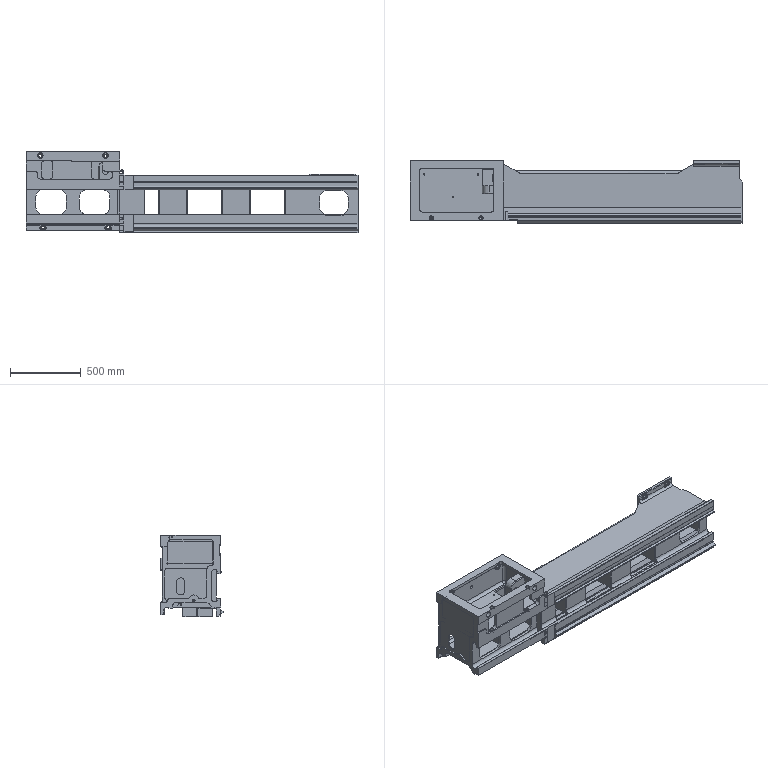Component | NX | LATHE_BED | 2 solids | 680 faces | volume 80560531 mm3 | plane 377 | cylinder 227 | cone 46 | torus 22 | sphere 8 | commonest cylinder face diameters 10 x65 40 x55 100 x27 50 x12 30 x11 20 x11 38 x10 22 x9